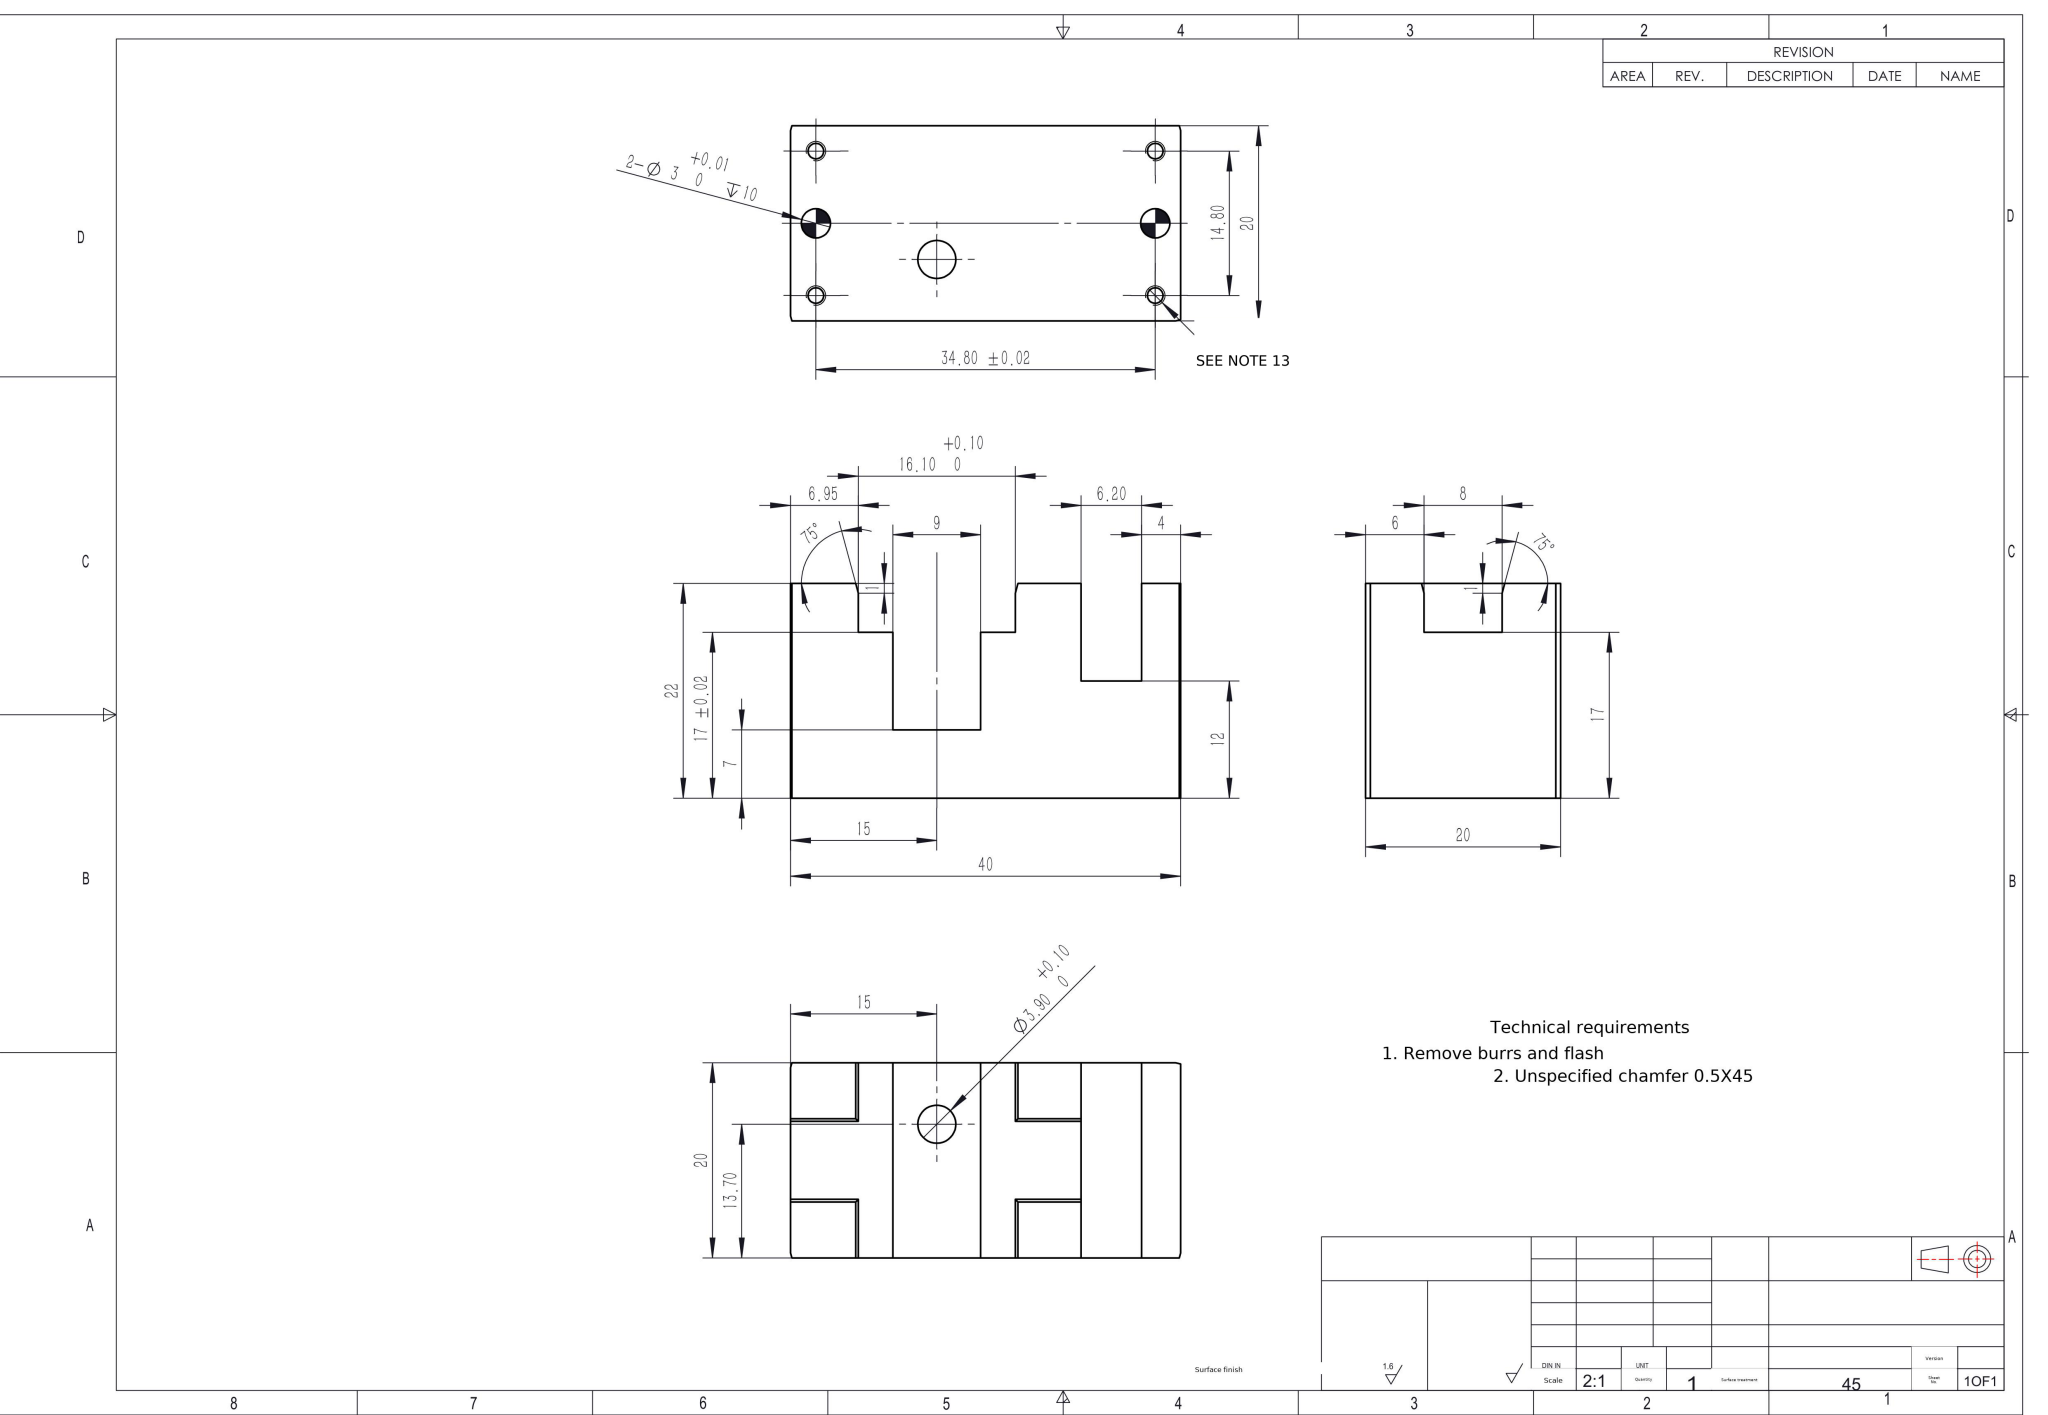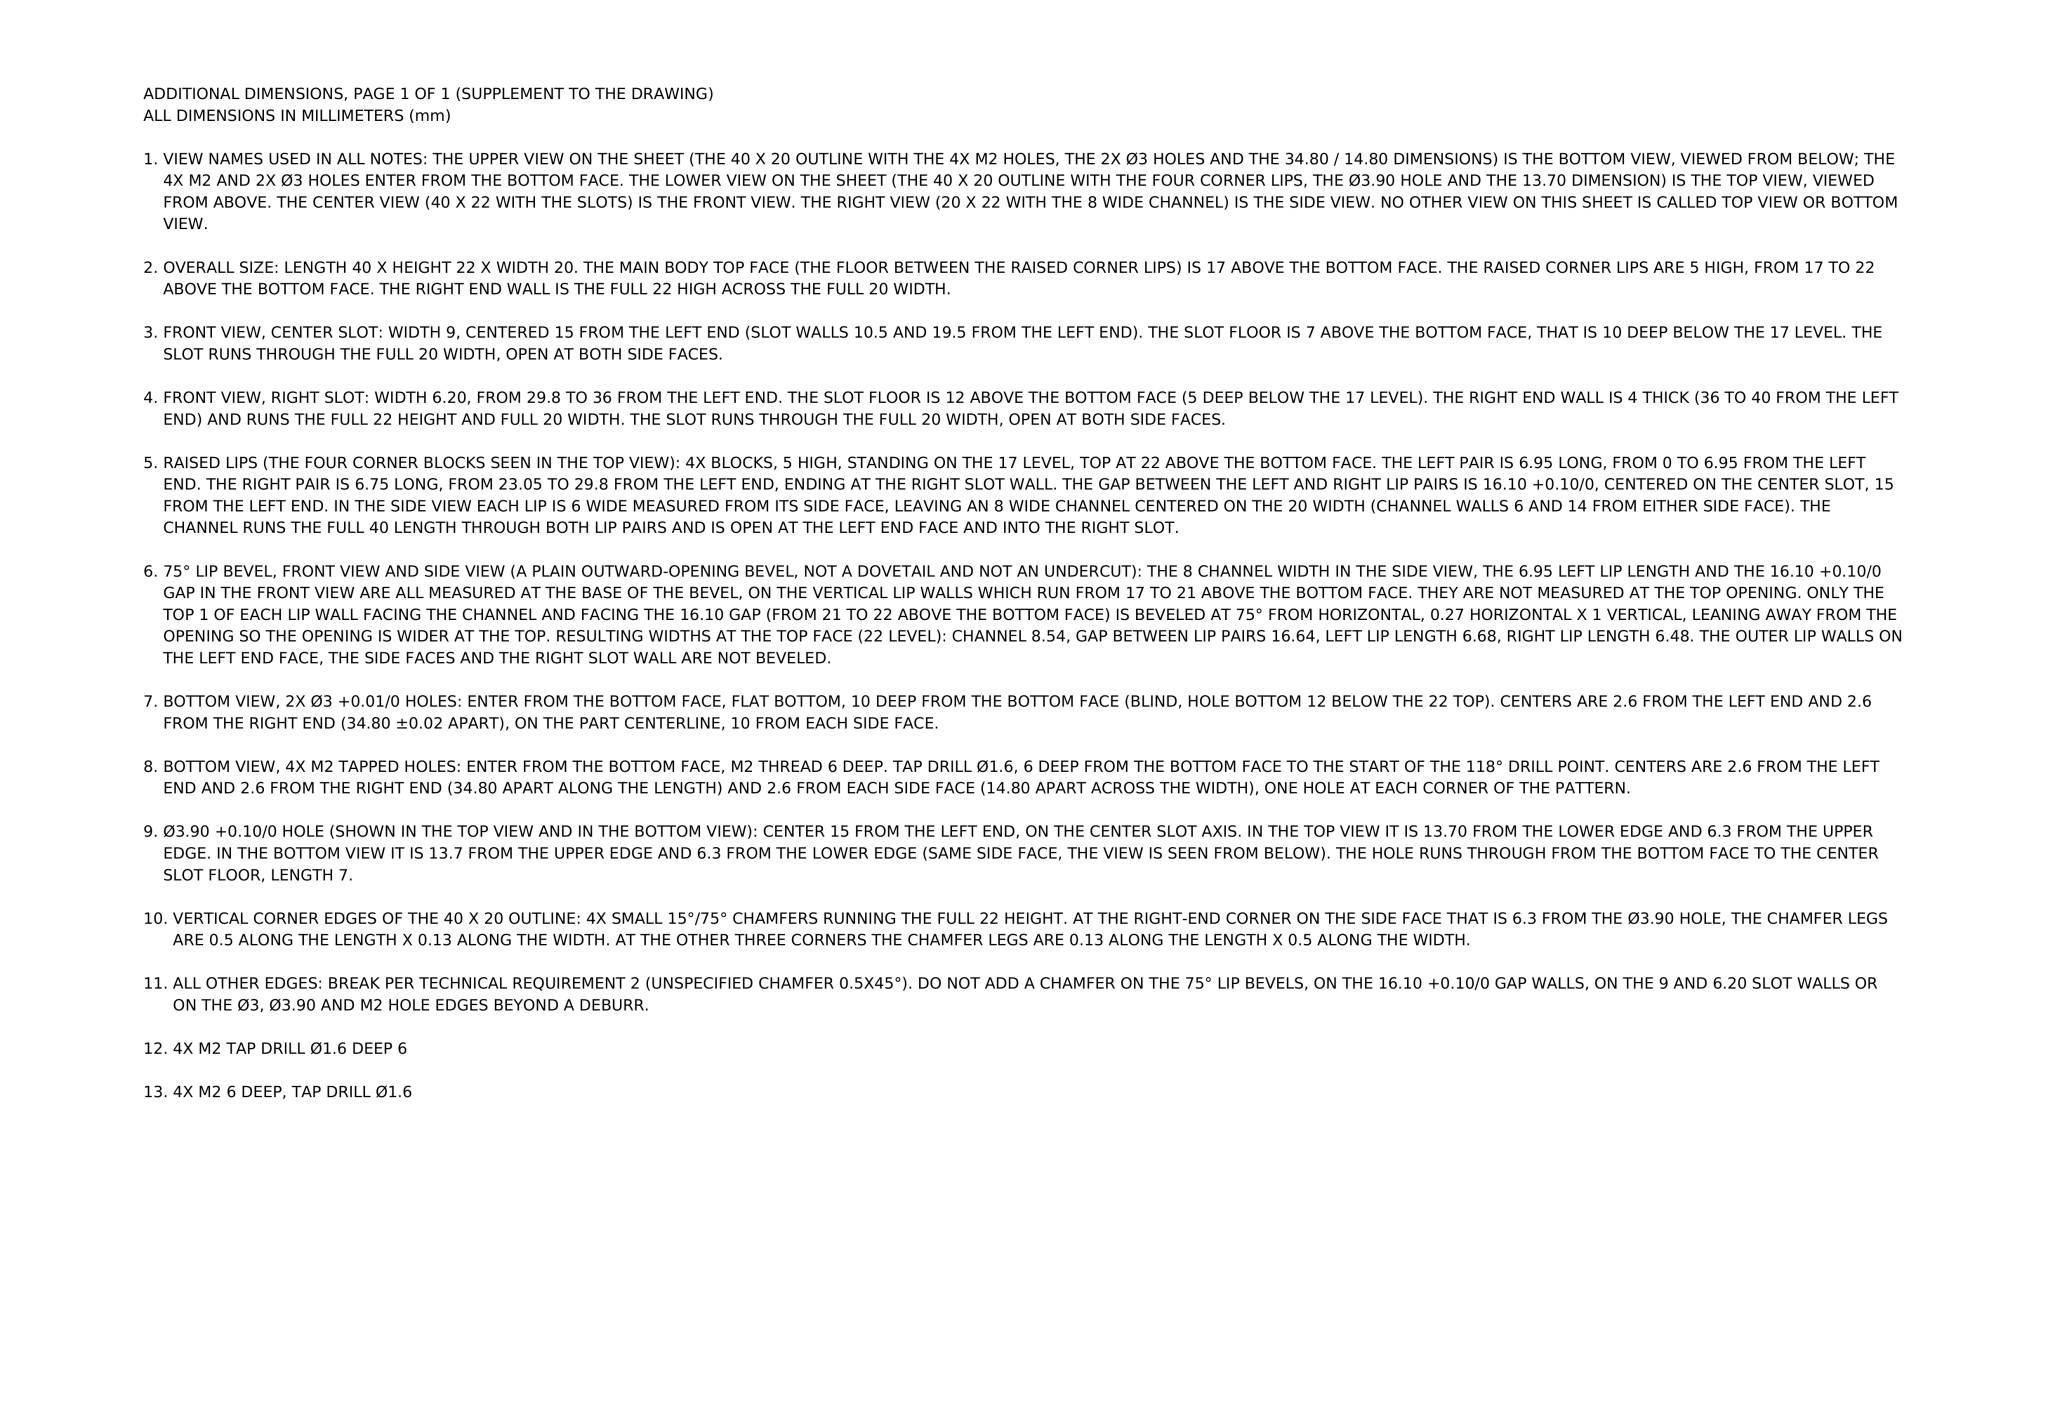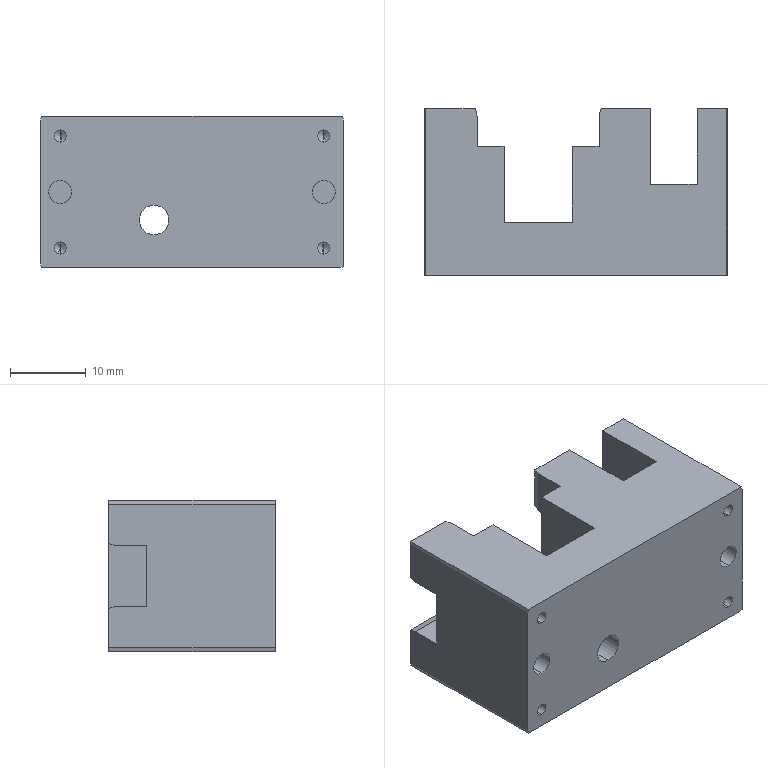Part | NX | mm | 1 solid | 62 faces | box 40 x 22 x 20 mm | volume 12118 mm3 | plane 40 | cylinder 14 | cone 8 | commonest cylinder face diameters 1.6 x8 3 x4 3.9 x2